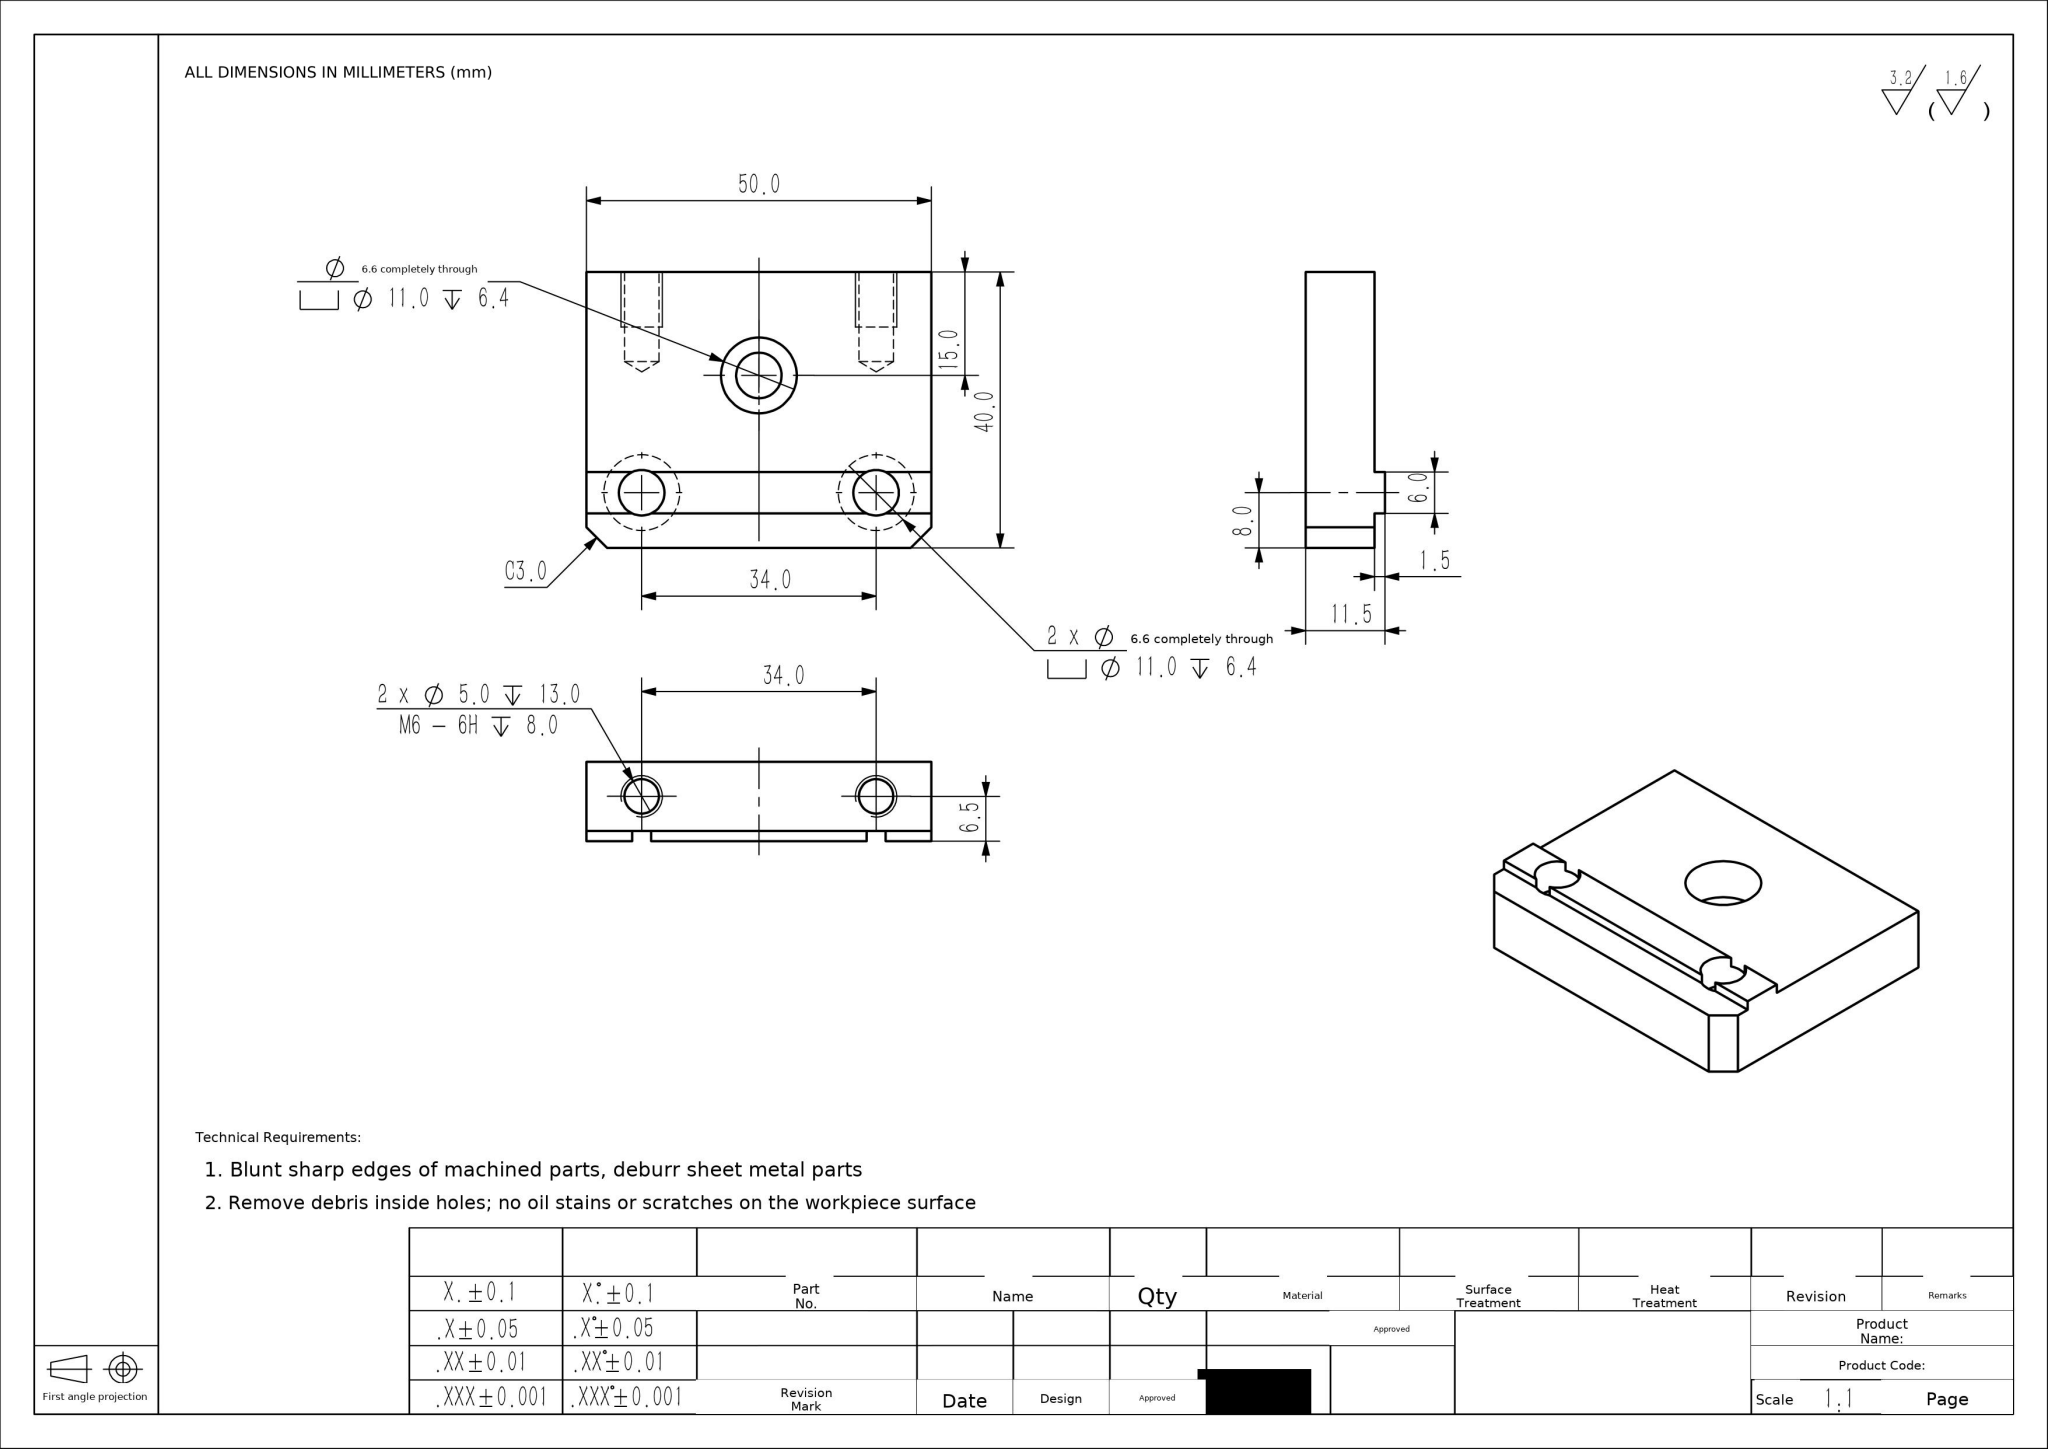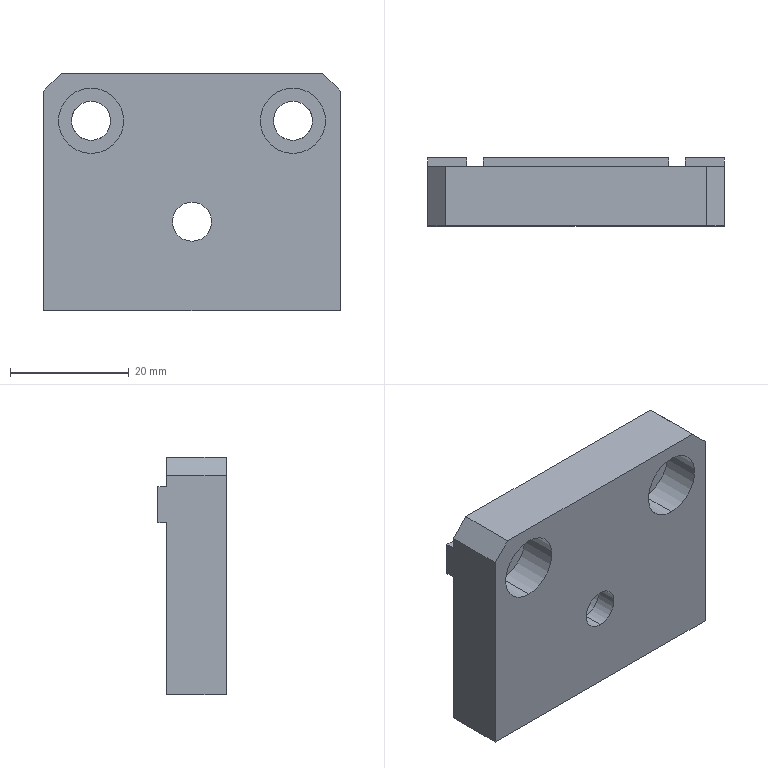Part | NX | mm | 1 solid | 41 faces | box 50 x 11.5 x 40 mm | volume 17536 mm3 | plane 21 | cylinder 16 | cone 4 | commonest cylinder face diameters 11 x6 6.6 x6 5 x4